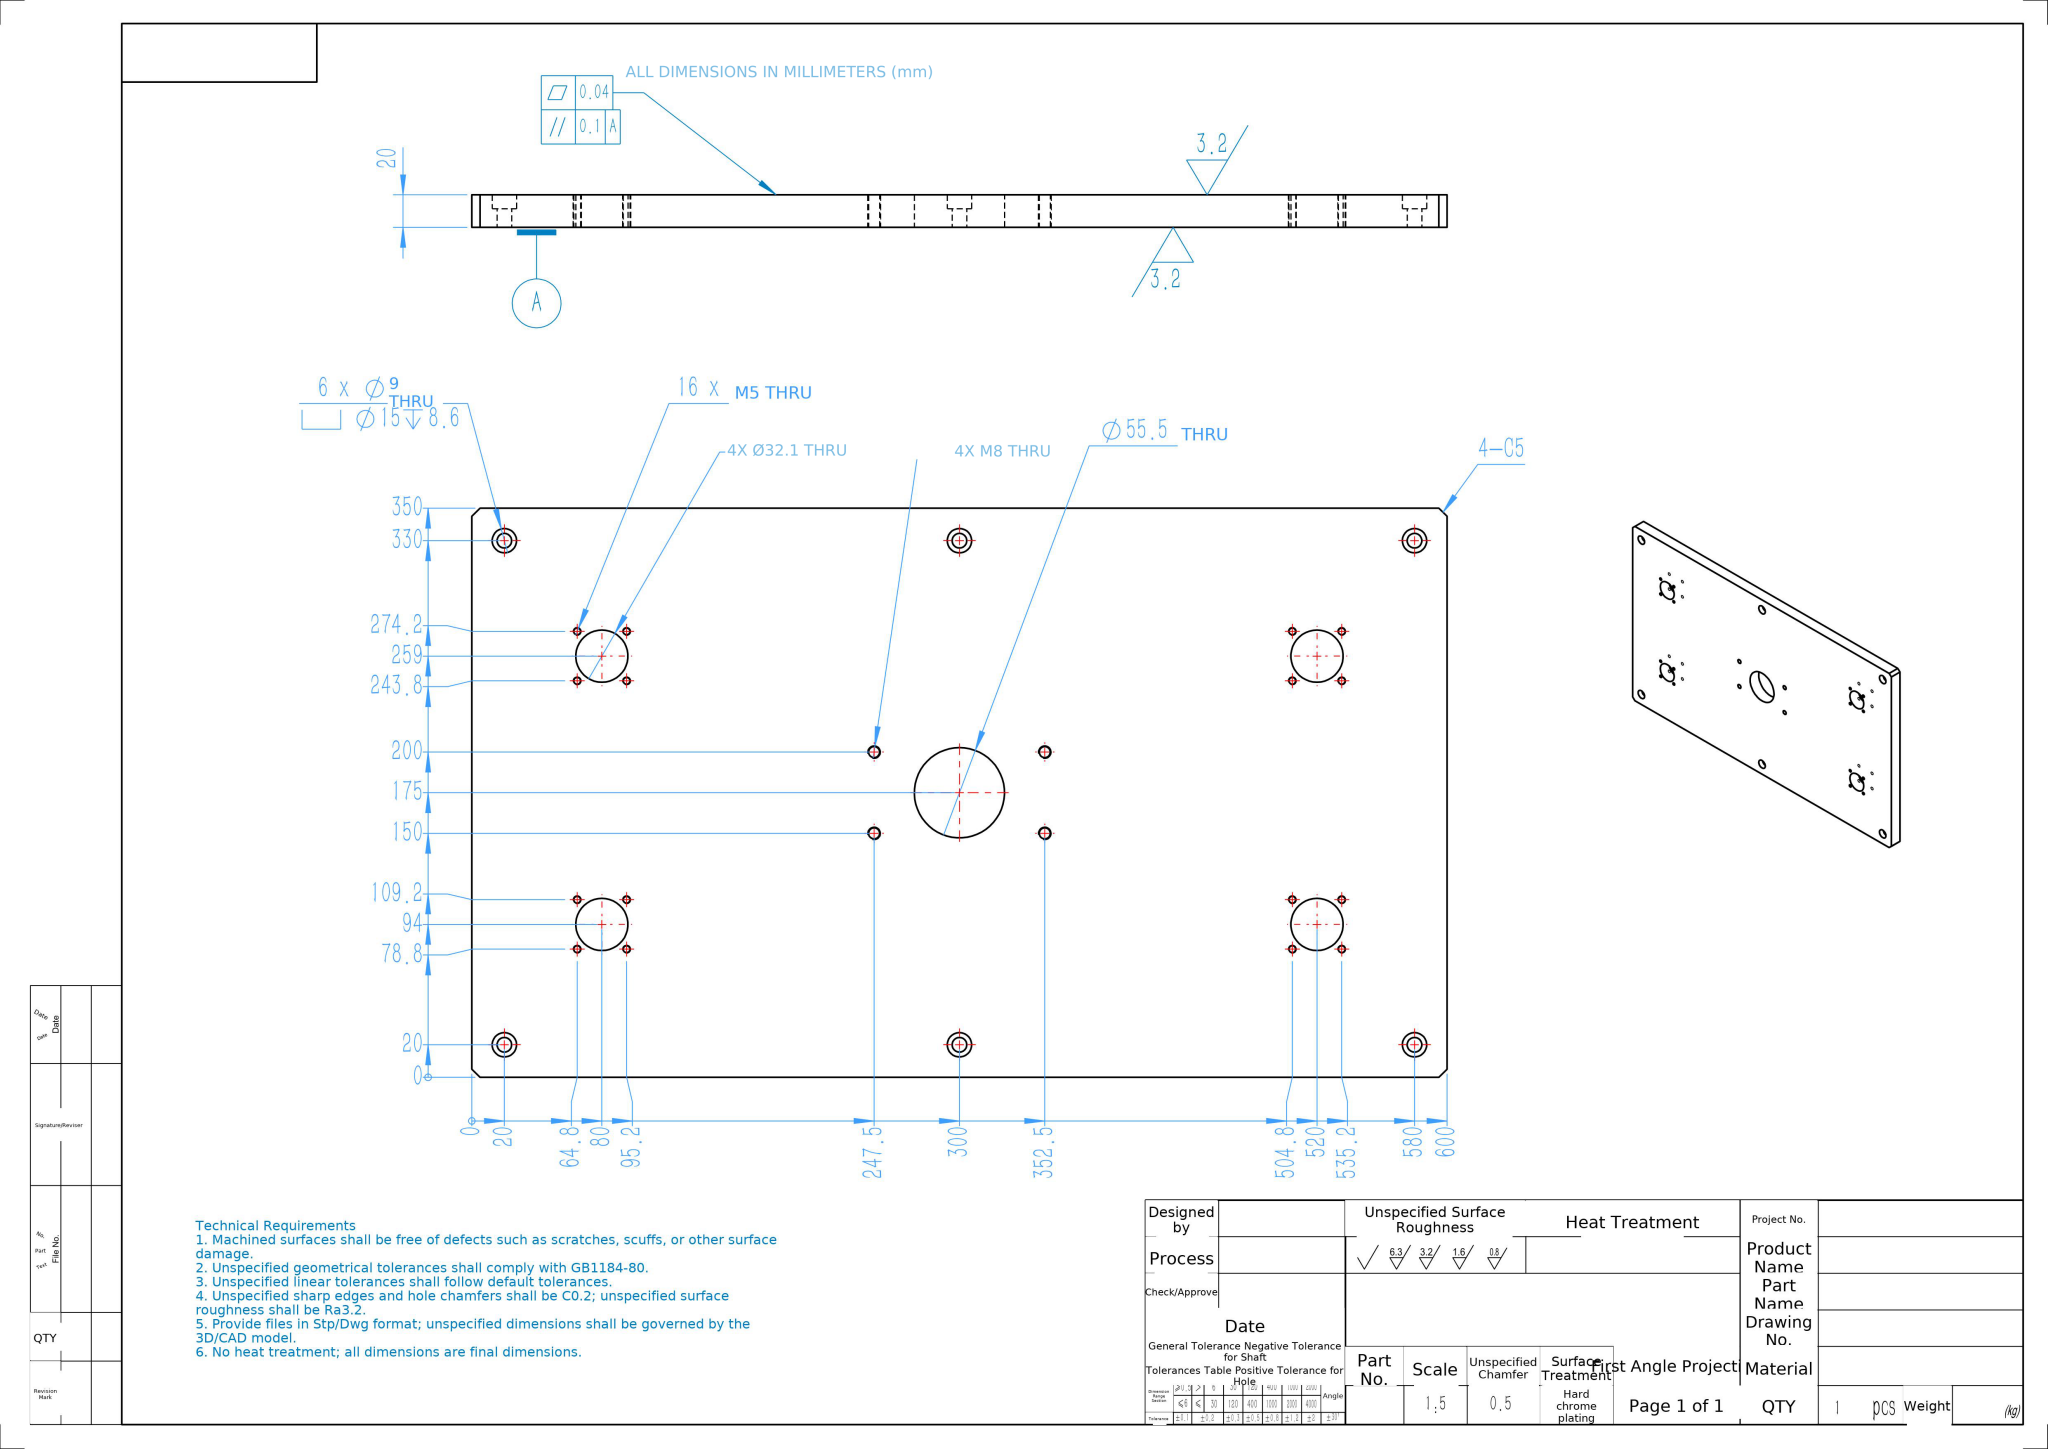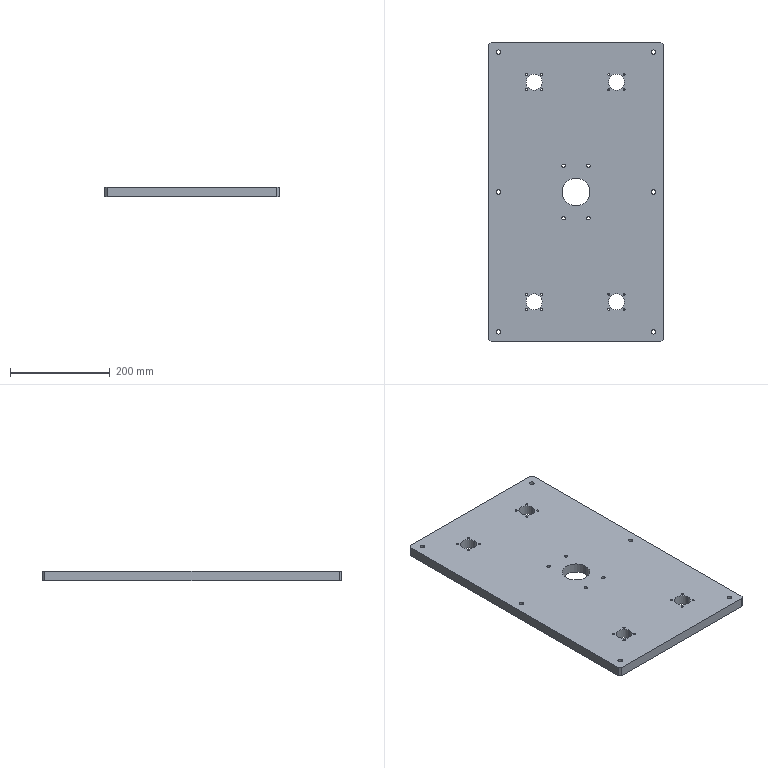Part | NX | mm | 1 solid | 90 faces | box 350 x 600 x 20 mm | volume 4065064 mm3 | cylinder 74 | plane 16 | commonest cylinder face diameters 4.2 x32 15 x12 9 x12 32.1 x8 6.8 x8 55.5 x2